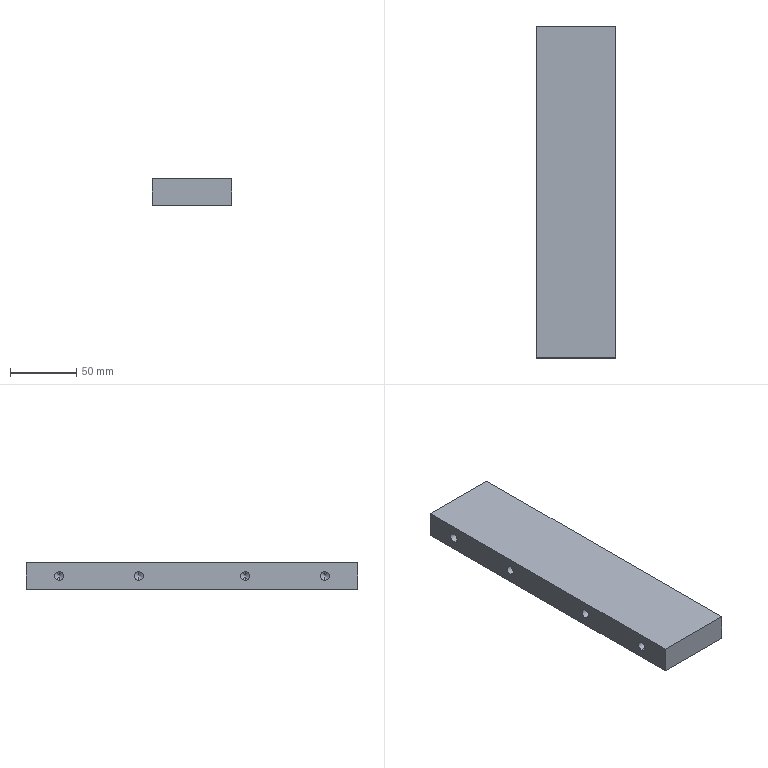Component | SolidWorks | F7-2 | 1 solid | 38 faces | box 60 x 250 x 20 mm | volume 293991 mm3 | cylinder 16 | cone 16 | plane 6 | commonest cylinder face diameters 6.8 x16
build123d program:
from build123d import *

# Parameters (mm, degrees)
SKETCH1_W             = 20
SKETCH1_H             = 250
BOSS_EXTRUDE1_DEPTH   = 60
M8_TAPPED_HOLE1_D     = 6.8
M8_TAPPED_HOLE1_DEPTH = 20
M8_TAPPED_HOLE1_TIP   = 2.043
M8_TAPPED_HOLE2_D     = 6.8
M8_TAPPED_HOLE2_DEPTH = 20
M8_TAPPED_HOLE2_TIP   = 2.043


with BuildPart() as part:
    # Sketch1 → Boss-Extrude1 (new body)
    with BuildSketch(Plane.XY):
        with Locations((127, 588)):
            Rectangle(SKETCH1_W, SKETCH1_H)
    extrude(amount=BOSS_EXTRUDE1_DEPTH)

    # M8 Tapped Hole1
    with Locations(Plane(origin=(0, 0, 0), x_dir=(-1, 0, 0), z_dir=(0, 0, -1))):
        with Locations((-127, 688), (-127, 628), (-127, 548), (-127, 488)):
            Hole(M8_TAPPED_HOLE1_D / 2, depth=M8_TAPPED_HOLE1_DEPTH)
            with Locations((0, 0, -(M8_TAPPED_HOLE1_DEPTH + M8_TAPPED_HOLE1_TIP / 2))):  # 118° drill point
                Cone(0, M8_TAPPED_HOLE1_D / 2, M8_TAPPED_HOLE1_TIP, mode=Mode.SUBTRACT)

    # M8 Tapped Hole2
    with Locations(Plane.XY.offset(60)):
        with Locations((127, 688), (127, 628), (127, 548), (127, 488)):
            Hole(M8_TAPPED_HOLE2_D / 2, depth=M8_TAPPED_HOLE2_DEPTH)
            with Locations((0, 0, -(M8_TAPPED_HOLE2_DEPTH + M8_TAPPED_HOLE2_TIP / 2))):  # 118° drill point
                Cone(0, M8_TAPPED_HOLE2_D / 2, M8_TAPPED_HOLE2_TIP, mode=Mode.SUBTRACT)


solid = part.part

# Placed as in the assembly
solid = solid.moved(Location((18, -599.721, 142), (0, 90, 0)))